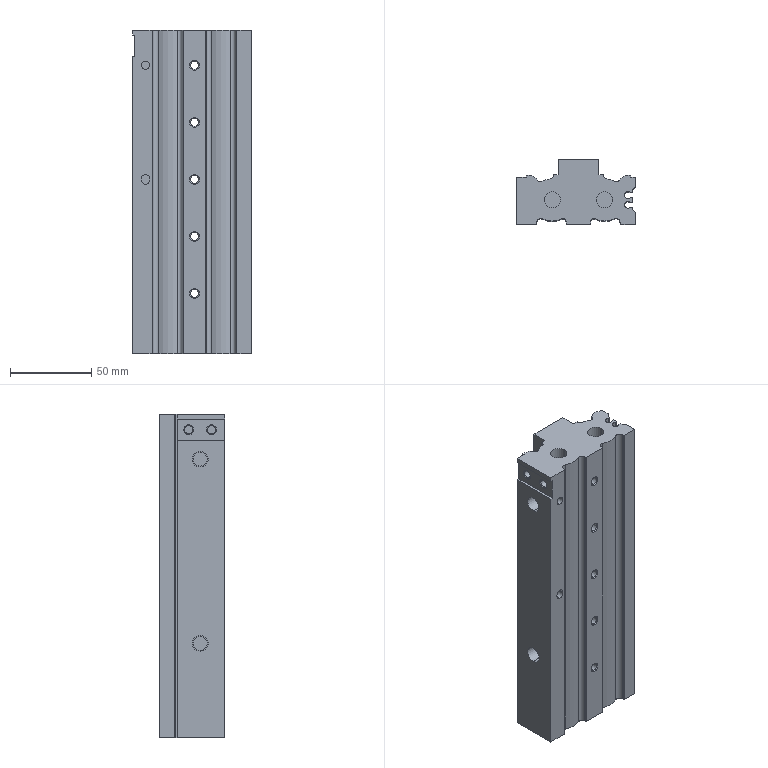Component | SolidWorks | SMC-MXS20-100AS-M9N-1_0SMC-MXS20-100AS-M9N-2-1 | 1 solid | 189 faces | box 73 x 40 x 198.5 mm | volume 356188 mm3 | cylinder 89 | plane 74 | cone 26 | commonest cylinder face diameters 4.917 x14 4.134 x12 5.1 x10 9.5 x10 5 x7 4 x6 8.566 x4 9.728 x4
build123d program:
from build123d import *

# Parameters (mm, degrees)
BOSS_EXTRUDE1_DEPTH            = 198.5
CUT_EXTRUDE1_DEPTH             = 198.5
CUT_EXTRUDE2_DEPTH             = 198.5
CUT_EXTRUDE3_DEPTH             = 198.5
CUT_EXTRUDE4_DEPTH             = 198.5
CUT_EXTRUDE5_DEPTH             = 198.5
CUT_EXTRUDE6_DEPTH             = 5
SKETCH8_R                      = 2.5
CUT_EXTRUDE7_DEPTH             = 5
LPATTERN1_COUNT                = 3
LPATTERN1_PITCH                = 30
LPATTERN1_COUNT_DIR2           = 2
LPATTERN1_PITCH_DIR2           = 18
SKETCH20_W                     = 1.5
SKETCH20_H                     = 13
CUT_EXTRUDE8_DEPTH             = 29
SKETCH23_R                     = 11
CUT_EXTRUDE9_DEPTH             = 1
SKETCH24_R                     = 11
CUT_EXTRUDE10_DEPTH            = 1
RC1_8_THREADMAJOR_SKETCH_R     = 4.864
RC1_8_THREADMAJOR_RELIEF_DEPTH = 6.5


with BuildPart() as part:
    # Sketch1 → Boss-Extrude1 (new body)
    with BuildSketch(Plane.XY):
        Polygon((-38, 0), (35, 0), (35, 29), (32, 29), (32, 30.5), (12.5, 30.5), (12.5, 40), (-12.5, 40), (-12.5, 30.5), (-32, 30.5), (-32, 29), (-38, 29), align=None)
    extrude(amount=BOSS_EXTRUDE1_DEPTH)

    # Sketch2 → Cut-Extrude1 (cut)
    with BuildSketch(Plane.XY):
        with BuildLine():
            Line((31.66, 10.4), (35, 10.4))
            Line((35, 10.4), (35, 13.6))
            Line((35, 13.6), (31.66, 13.6))
            ThreePointArc((31.66, 13.6), (28.2, 12), (31.66, 10.4))
        make_face()
    extrude(amount=CUT_EXTRUDE1_DEPTH, mode=Mode.SUBTRACT)

    # Sketch3 → Cut-Extrude2 (cut)
    with BuildSketch(Plane.XY):
        with BuildLine():
            Line((31.66, 16.4), (35, 16.4))
            Line((35, 16.4), (35, 19.6))
            Line((35, 19.6), (31.66, 19.6))
            ThreePointArc((31.66, 19.6), (28.2, 18), (31.66, 16.4))
        make_face()
    extrude(amount=CUT_EXTRUDE2_DEPTH, mode=Mode.SUBTRACT)

    # Sketch4 → Cut-Extrude3 (cut)
    with BuildSketch(Plane.XY):
        with BuildLine():
            Line((-26.001, -2), (26.001, -2))
            Line((26.001, -2), (26.001, 0))
            Line((26.001, 0), (25.501, 0.5))
            Line((25.501, 0.5), (25.501, 1.171))
            ThreePointArc((25.501, 1.171), (24.31, 3.301), (21.872, 3.401))
            ThreePointArc((21.872, 3.401), (16.133, 2.001), (10.367, 3.284))
            ThreePointArc((10.367, 3.284), (8.436, 3.175), (7.5, 1.482))
            Line((7.5, 1.482), (7.5, 0.5))
            Line((7.5, 0.5), (7, 0))
            Line((7, 0), (-7, 0))
            Line((-7, 0), (-7.5, 0.5))
            Line((-7.5, 0.5), (-7.5, 1.482))
            ThreePointArc((-7.5, 1.482), (-8.436, 3.175), (-10.367, 3.284))
            ThreePointArc((-10.367, 3.284), (-16.133, 2.001), (-21.872, 3.401))
            ThreePointArc((-21.872, 3.401), (-24.31, 3.301), (-25.501, 1.171))
            Line((-25.501, 1.171), (-25.501, 0.5))
            Line((-25.501, 0.5), (-26.001, 0))
            Line((-26.001, 0), (-26.001, -2))
        make_face()
    extrude(amount=CUT_EXTRUDE3_DEPTH, mode=Mode.SUBTRACT)

    # Sketch5 → Cut-Extrude4 (cut)
    with BuildSketch(Plane.XY):
        with BuildLine():
            Line((-38, 30), (-30.3, 30))
            ThreePointArc((-30.3, 30), (-27.318, 29.207), (-25.125, 27.036))
            ThreePointArc((-25.125, 27.036), (-23.918, 26.116), (-22.413, 26.308))
            ThreePointArc((-22.413, 26.308), (-19.941, 27.388), (-17.3, 27.935))
            ThreePointArc((-17.3, 27.935), (-16.017, 28.583), (-15.5, 29.925))
            Line((-15.5, 29.925), (-15.5, 40))
            Line((-15.5, 40), (15.5, 40))
            Line((15.5, 40), (15.5, 29.925))
            ThreePointArc((15.5, 29.925), (16.017, 28.583), (17.3, 27.935))
            ThreePointArc((17.3, 27.935), (19.941, 27.388), (22.413, 26.308))
            ThreePointArc((22.413, 26.308), (23.918, 26.116), (25.125, 27.036))
            ThreePointArc((25.125, 27.036), (27.318, 29.207), (30.3, 30))
            Line((30.3, 30), (38, 30))
            Line((38, 30), (38, 42))
            Line((38, 42), (-38, 42))
            Line((-38, 42), (-38, 30))
        make_face()
    extrude(amount=CUT_EXTRUDE4_DEPTH, mode=Mode.SUBTRACT)

    # Sketch6 → Cut-Extrude5 (cut)
    with BuildSketch(Plane.XY):
        Polygon((33.1, 8.9), (35, 7), (35, 23), (33.1, 21.1), align=None)
    extrude(amount=CUT_EXTRUDE5_DEPTH, mode=Mode.SUBTRACT)

    # Sketch7 → Cut-Extrude6 (cut)
    with BuildSketch(Plane(origin=(0, 0, 0), x_dir=(1, 0, 0), z_dir=(0, 1, 0))):
        with BuildLine():
            Line((-32.5, -106.5), (-32.5, -107.5))
            ThreePointArc((-32.5, -107.5), (-30, -110), (-27.5, -107.5))
            Line((-27.5, -107.5), (-27.5, -106.5))
            ThreePointArc((-27.5, -106.5), (-30, -104), (-32.5, -106.5))
        make_face()
    extrude(amount=CUT_EXTRUDE6_DEPTH, mode=Mode.SUBTRACT)

    # Sketch8 → Cut-Extrude7 (cut)
    with BuildSketch(Plane(origin=(0, 0, 0), x_dir=(1, 0, 0), z_dir=(0, 1, 0))):
        with Locations(Location((-30, -177, 0), (0, 0, 270))):
            Circle(SKETCH8_R)
    extrude(amount=CUT_EXTRUDE7_DEPTH, mode=Mode.SUBTRACT)

    # Sketch9 → Cut-Revolve1 (revolve, cut)
    with BuildSketch(Plane.XY.offset(37), mode=Mode.PRIVATE) as cut_revolve1_sk:
        Polygon((0, 40.5), (4.75, 40.5), (4.75, 29), (2.55, 29), (2.55, 12), (2.458, 12), (2.458, 0.5415), (3, 0), (0, 0), align=None)
    revolve(cut_revolve1_sk.sketch.rotate(Axis((0, 0, 37), (0, 1, 0)), 270), axis=Axis((0, 0, 37), (0, 1, 0)), mode=Mode.SUBTRACT)

    # Sketch10 → Cut-Revolve2 (revolve, cut)
    with BuildSketch(Plane.XY.offset(177), mode=Mode.PRIVATE) as cut_revolve2_sk:
        Polygon((0, 40.5), (4.75, 40.5), (4.75, 29), (2.55, 29), (2.55, 12), (2.458, 12), (2.458, 0.5415), (3, 0), (0, 0), align=None)
    revolve(cut_revolve2_sk.sketch.rotate(Axis((0, 0, 177), (0, 1, 0)), 270), axis=Axis((0, 0, 177), (0, 1, 0)), mode=Mode.SUBTRACT)

    # Sketch11 → Cut-Revolve3 (revolve, cut)
    with BuildSketch(Plane.XY.offset(142), mode=Mode.PRIVATE) as cut_revolve3_sk:
        Polygon((0, 40.5), (4.75, 40.5), (4.75, 29), (2.55, 29), (2.55, 12), (2.458, 12), (2.458, 0.5415), (3, 0), (0, 0), align=None)
    revolve(cut_revolve3_sk.sketch.rotate(Axis((0, 0, 142), (0, 1, 0)), 270), axis=Axis((0, 0, 142), (0, 1, 0)), mode=Mode.SUBTRACT)

    # Sketch12 → Cut-Revolve4 (revolve, cut)
    with BuildSketch(Plane.XY.offset(107), mode=Mode.PRIVATE) as cut_revolve4_sk:
        Polygon((0, 40.5), (4.75, 40.5), (4.75, 29), (2.55, 29), (2.55, 12), (2.458, 12), (2.458, 0.5415), (3, 0), (0, 0), align=None)
    revolve(cut_revolve4_sk.sketch.rotate(Axis((0, 0, 107), (0, 1, 0)), 270), axis=Axis((0, 0, 107), (0, 1, 0)), mode=Mode.SUBTRACT)

    # Sketch13 → Cut-Revolve5 (revolve, cut)
    with BuildSketch(Plane.XY.offset(72), mode=Mode.PRIVATE) as cut_revolve5_sk:
        Polygon((0, 40.5), (4.75, 40.5), (4.75, 29), (2.55, 29), (2.55, 12), (2.458, 12), (2.458, 0.5415), (3, 0), (0, 0), align=None)
    revolve(cut_revolve5_sk.sketch.rotate(Axis((0, 0, 72), (0, 1, 0)), 270), axis=Axis((0, 0, 72), (0, 1, 0)), mode=Mode.SUBTRACT)

    # Sketch14 → Cut-Revolve6 (revolve, cut)
    with BuildSketch(Plane.XY.offset(58), mode=Mode.PRIVATE) as cut_revolve6_sk:
        Polygon((-38, 15), (-38, 19.864), (-37.419, 19.283), (-28.272, 19.283), (-28.272, 15), align=None)
    revolve(cut_revolve6_sk.sketch.rotate(Axis((-28.272, 15, 58), (-1, 0, 0)), 270), axis=Axis((-28.272, 15, 58), (-1, 0, 0)), mode=Mode.SUBTRACT)

    # Sketch15 → Cut-Revolve7 (revolve, cut)
    with BuildSketch(Plane.XY.offset(171), mode=Mode.PRIVATE) as cut_revolve7_sk:
        Polygon((-38, 15), (-38, 19.864), (-37.419, 19.283), (-28.272, 19.283), (-28.272, 15), align=None)
    revolve(cut_revolve7_sk.sketch.rotate(Axis((-28.272, 15, 171), (-1, 0, 0)), 270), axis=Axis((-28.272, 15, 171), (-1, 0, 0)), mode=Mode.SUBTRACT)

    # Sketch16 → Cut-Revolve8 (revolve, cut)
    with BuildSketch(Plane(origin=(-30, 0, 0), x_dir=(0, 0, -1), z_dir=(1, 0, 0)), mode=Mode.PRIVATE) as cut_revolve8_sk:
        Polygon((-8, 6), (-8, 8.067), (-0.433, 8.067), (0, 8.5), (0, 6), align=None)
    cut_revolve8 = revolve(cut_revolve8_sk.sketch.rotate(Axis((-30, 6, 0), (0, 0, 1)), 270), axis=Axis((-30, 6, 0), (0, 0, 1)), mode=Mode.SUBTRACT)

    # LPattern1: Cut-Revolve8 3 × 2
    with Locations(*[(i * LPATTERN1_PITCH, j * LPATTERN1_PITCH_DIR2, 0) for i in range(LPATTERN1_COUNT) for j in range(LPATTERN1_COUNT_DIR2) if (i, j) != (0, 0)]):
        add(cut_revolve8, mode=Mode.SUBTRACT)

    # Sketch18 → Cut-Revolve9 (revolve, cut)
    with BuildSketch(Plane(origin=(0, 15, 0), x_dir=(1, 0, 0), z_dir=(0, 1, 0)), mode=Mode.PRIVATE) as cut_revolve9_sk:
        Polygon((-16, -198.5), (-21, -198.5), (-21, -149.25), (-26, -149.25), (-26, -46.25), (-16, -46.25), align=None)
    revolve(cut_revolve9_sk.sketch.rotate(Axis((-16, 15, 46.25), (0, 0, 1)), 180), axis=Axis((-16, 15, 46.25), (0, 0, 1)), mode=Mode.SUBTRACT)

    # Sketch19 → Cut-Revolve10 (revolve, cut)
    with BuildSketch(Plane(origin=(0, 15, 0), x_dir=(1, 0, 0), z_dir=(0, 1, 0)), mode=Mode.PRIVATE) as cut_revolve10_sk:
        Polygon((16, -198.5), (11, -198.5), (11, -149.25), (6, -149.25), (6, -46.25), (16, -46.25), align=None)
    revolve(cut_revolve10_sk.sketch.rotate(Axis((16, 15, 46.25), (0, 0, 1)), 180), axis=Axis((16, 15, 46.25), (0, 0, 1)), mode=Mode.SUBTRACT)

    # Sketch20 → Cut-Extrude8 (cut)
    with BuildSketch(Plane(origin=(0, 0, 0), x_dir=(1, 0, 0), z_dir=(0, 1, 0))):
        with Locations((-37.25, -189)):
            Rectangle(SKETCH20_W, SKETCH20_H)
    extrude(amount=CUT_EXTRUDE8_DEPTH, mode=Mode.SUBTRACT)

    # Sketch21 → Cut-Revolve11 (revolve, cut)
    with BuildSketch(Plane(origin=(0, 8, 0), x_dir=(1, 0, 0), z_dir=(0, 1, 0)), mode=Mode.PRIVATE) as cut_revolve11_sk:
        Polygon((-30, -189), (-30, -191.458), (-35.959, -191.458), (-36.5, -192), (-36.5, -189), align=None)
    revolve(cut_revolve11_sk.sketch.rotate(Axis((-36.5, 8, 189), (1, 0, 0)), 180), axis=Axis((-36.5, 8, 189), (1, 0, 0)), mode=Mode.SUBTRACT)

    # Sketch22 → Cut-Revolve12 (revolve, cut)
    with BuildSketch(Plane(origin=(0, 22, 0), x_dir=(1, 0, 0), z_dir=(0, 1, 0)), mode=Mode.PRIVATE) as cut_revolve12_sk:
        Polygon((-30, -189), (-30, -191.458), (-35.959, -191.458), (-36.5, -192), (-36.5, -189), align=None)
    revolve(cut_revolve12_sk.sketch.rotate(Axis((-36.5, 22, 189), (1, 0, 0)), 180), axis=Axis((-36.5, 22, 189), (1, 0, 0)), mode=Mode.SUBTRACT)

    # Sketch23 → Cut-Extrude9 (cut)
    with BuildSketch(Plane.XY):
        with Locations((-16, 15)):
            Circle(SKETCH23_R)
    extrude(amount=CUT_EXTRUDE9_DEPTH, mode=Mode.SUBTRACT)

    # Sketch24 → Cut-Extrude10 (cut)
    with BuildSketch(Plane.XY):
        with Locations((16, 15)):
            Circle(SKETCH24_R)
    extrude(amount=CUT_EXTRUDE10_DEPTH, mode=Mode.SUBTRACT)

    # Rc1-8_ThreadMajor_Sketch → Rc1-8_ThreadMajor_Relief (cut)
    with BuildSketch(Plane.ZY.offset(38)):
        with Locations((58, 15)):
            Circle(RC1_8_THREADMAJOR_SKETCH_R)
        with Locations((171, 15)):
            Circle(RC1_8_THREADMAJOR_SKETCH_R)
    extrude(amount=-RC1_8_THREADMAJOR_RELIEF_DEPTH, mode=Mode.SUBTRACT)


solid = part.part

# Placed as in the assembly
solid = solid.moved(Location((-235.009, 50.721, -54.911), (0, 0, 0)))